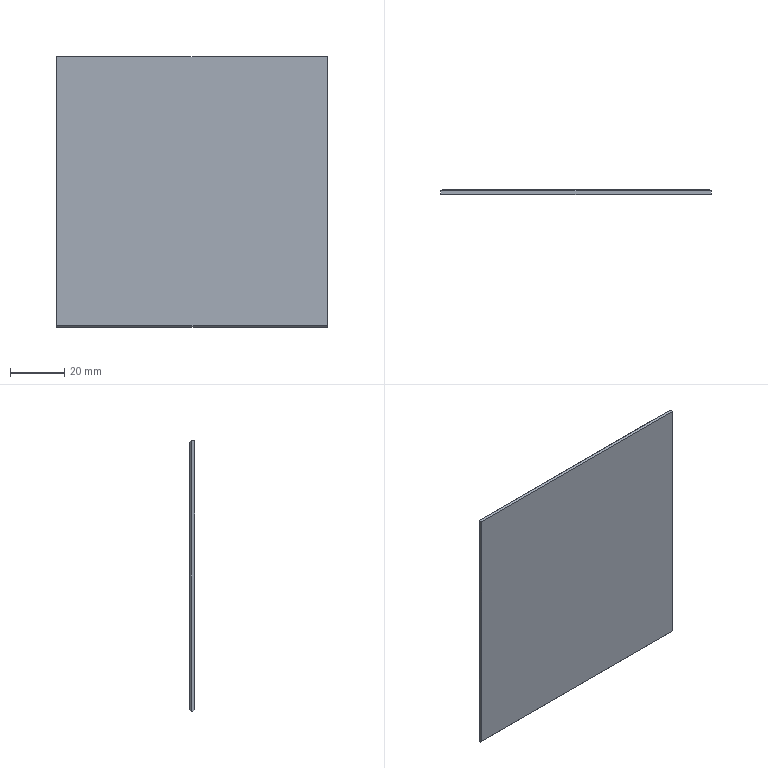Component | SolidWorks | PC-CAJ-P08-1_PM-CAJ-P60-1 | 1 solid | 11 faces | box 100 x 1.9 x 100 mm | volume 18910 mm3 | plane 11 | material Plain Carbon Steel
STEP:
#1=COLOUR_RGB('',0.7922,0.8196,0.9333);
#2=FILL_AREA_STYLE_COLOUR('',#1);
#3=FILL_AREA_STYLE('',(#2));
#4=SURFACE_STYLE_FILL_AREA(#3);
#5=SURFACE_SIDE_STYLE('',(#4));
#6=SURFACE_STYLE_USAGE(.BOTH.,#5);
#7=PRESENTATION_STYLE_ASSIGNMENT((#6));
#8=CARTESIAN_POINT('',(13.181,-26.622,8.976));
#9=VERTEX_POINT('',#8);
#10=CARTESIAN_POINT('',(13.181,-26.622,5.063));
#11=VERTEX_POINT('',#10);
#12=CARTESIAN_POINT('',(13.181,-26.622,7.008));
#13=DIRECTION('',(-0.,-0.,-1.));
#14=VECTOR('',#13,39.37);
#15=LINE('',#12,#14);
#16=EDGE_CURVE('',#9,#11,#15,.T.);
#17=ORIENTED_EDGE('',*,*,#16,.T.);
#18=CARTESIAN_POINT('',(13.181,-26.598,5.039));
#19=VERTEX_POINT('',#18);
#20=CARTESIAN_POINT('',(13.181,-28.579,7.02));
#21=DIRECTION('',(0.,0.7071,-0.7071));
#22=VECTOR('',#21,39.37);
#23=LINE('',#20,#22);
#24=EDGE_CURVE('',#11,#19,#23,.T.);
#25=ORIENTED_EDGE('',*,*,#24,.T.);
#26=CARTESIAN_POINT('',(13.181,-26.571,5.039));
#27=VERTEX_POINT('',#26);
#28=CARTESIAN_POINT('',(13.181,-26.585,5.039));
#29=DIRECTION('',(0.,1.,-0.));
#30=VECTOR('',#29,39.37);
#31=LINE('',#28,#30);
#32=EDGE_CURVE('',#19,#27,#31,.T.);
#33=ORIENTED_EDGE('',*,*,#32,.T.);
#34=CARTESIAN_POINT('',(13.181,-26.571,8.976));
#35=VERTEX_POINT('',#34);
#36=CARTESIAN_POINT('',(13.181,-26.571,8.976));
#37=DIRECTION('',(0.,0.,1.));
#38=VECTOR('',#37,39.37);
#39=LINE('',#36,#38);
#40=EDGE_CURVE('',#27,#35,#39,.T.);
#41=ORIENTED_EDGE('',*,*,#40,.T.);
#42=CARTESIAN_POINT('',(13.181,-26.585,8.976));
#43=DIRECTION('',(-0.,-1.,0.));
#44=VECTOR('',#43,39.37);
#45=LINE('',#42,#44);
#46=EDGE_CURVE('',#35,#9,#45,.T.);
#47=ORIENTED_EDGE('',*,*,#46,.T.);
#48=EDGE_LOOP('',(#17,#25,#33,#41,#47));
#49=FACE_OUTER_BOUND('',#48,.T.);
#50=CARTESIAN_POINT('',(13.181,-26.622,8.976));
#51=DIRECTION('',(1.,-0.,-0.));
#52=DIRECTION('',(-0.,-0.,-1.));
#53=AXIS2_PLACEMENT_3D('',#50,#51,#52);
#54=PLANE('',#53);
#55=ADVANCED_FACE('',(#49),#54,.T.);
#56=ORIENTED_EDGE('',*,*,#32,.F.);
#57=CARTESIAN_POINT('',(9.244,-26.598,5.039));
#58=VERTEX_POINT('',#57);
#59=CARTESIAN_POINT('',(13.181,-26.598,5.039));
#60=DIRECTION('',(-1.,0.,0.));
#61=VECTOR('',#60,39.37);
#62=LINE('',#59,#61);
#63=EDGE_CURVE('',#19,#58,#62,.T.);
#64=ORIENTED_EDGE('',*,*,#63,.T.);
#65=CARTESIAN_POINT('',(9.244,-26.571,5.039));
#66=VERTEX_POINT('',#65);
#67=CARTESIAN_POINT('',(9.244,-26.585,5.039));
#68=DIRECTION('',(0.,1.,-0.));
#69=VECTOR('',#68,39.37);
#70=LINE('',#67,#69);
#71=EDGE_CURVE('',#58,#66,#70,.T.);
#72=ORIENTED_EDGE('',*,*,#71,.T.);
#73=CARTESIAN_POINT('',(13.181,-26.571,5.039));
#74=DIRECTION('',(1.,-0.,-0.));
#75=VECTOR('',#74,39.37);
#76=LINE('',#73,#75);
#77=EDGE_CURVE('',#66,#27,#76,.T.);
#78=ORIENTED_EDGE('',*,*,#77,.T.);
#79=EDGE_LOOP('',(#56,#64,#72,#78));
#80=FACE_OUTER_BOUND('',#79,.T.);
#81=CARTESIAN_POINT('',(13.181,-26.622,5.039));
#82=DIRECTION('',(-0.,-0.,-1.));
#83=DIRECTION('',(-1.,0.,0.));
#84=AXIS2_PLACEMENT_3D('',#81,#82,#83);
#85=PLANE('',#84);
#86=ADVANCED_FACE('',(#80),#85,.T.);
#87=CARTESIAN_POINT('',(9.244,-26.622,8.976));
#88=VERTEX_POINT('',#87);
#89=CARTESIAN_POINT('',(9.244,-26.622,5.063));
#90=VERTEX_POINT('',#89);
#91=CARTESIAN_POINT('',(9.244,-26.622,7.008));
#92=DIRECTION('',(-0.,-0.,-1.));
#93=VECTOR('',#92,39.37);
#94=LINE('',#91,#93);
#95=EDGE_CURVE('',#88,#90,#94,.T.);
#96=ORIENTED_EDGE('',*,*,#95,.T.);
#97=CARTESIAN_POINT('',(13.181,-26.622,5.063));
#98=DIRECTION('',(1.,-0.,-0.));
#99=VECTOR('',#98,39.37);
#100=LINE('',#97,#99);
#101=EDGE_CURVE('',#90,#11,#100,.T.);
#102=ORIENTED_EDGE('',*,*,#101,.T.);
#103=ORIENTED_EDGE('',*,*,#16,.F.);
#104=CARTESIAN_POINT('',(11.213,-26.622,8.976));
#105=DIRECTION('',(-1.,0.,0.));
#106=VECTOR('',#105,39.37);
#107=LINE('',#104,#106);
#108=EDGE_CURVE('',#9,#88,#107,.T.);
#109=ORIENTED_EDGE('',*,*,#108,.T.);
#110=EDGE_LOOP('',(#96,#102,#103,#109));
#111=FACE_OUTER_BOUND('',#110,.T.);
#112=CARTESIAN_POINT('',(13.181,-26.622,8.976));
#113=DIRECTION('',(-0.,-1.,0.));
#114=DIRECTION('',(-1.,0.,0.));
#115=AXIS2_PLACEMENT_3D('',#112,#113,#114);
#116=PLANE('',#115);
#117=ADVANCED_FACE('',(#111),#116,.T.);
#118=ORIENTED_EDGE('',*,*,#46,.F.);
#119=CARTESIAN_POINT('',(9.244,-26.571,8.976));
#120=VERTEX_POINT('',#119);
#121=CARTESIAN_POINT('',(9.244,-26.571,8.976));
#122=DIRECTION('',(-1.,0.,0.));
#123=VECTOR('',#122,39.37);
#124=LINE('',#121,#123);
#125=EDGE_CURVE('',#35,#120,#124,.T.);
#126=ORIENTED_EDGE('',*,*,#125,.T.);
#127=CARTESIAN_POINT('',(9.244,-26.585,8.976));
#128=DIRECTION('',(-0.,-1.,0.));
#129=VECTOR('',#128,39.37);
#130=LINE('',#127,#129);
#131=EDGE_CURVE('',#120,#88,#130,.T.);
#132=ORIENTED_EDGE('',*,*,#131,.T.);
#133=ORIENTED_EDGE('',*,*,#108,.F.);
#134=EDGE_LOOP('',(#118,#126,#132,#133));
#135=FACE_OUTER_BOUND('',#134,.T.);
#136=CARTESIAN_POINT('',(9.244,-26.622,8.976));
#137=DIRECTION('',(0.,0.,1.));
#138=DIRECTION('',(1.,-0.,-0.));
#139=AXIS2_PLACEMENT_3D('',#136,#137,#138);
#140=PLANE('',#139);
#141=ADVANCED_FACE('',(#135),#140,.T.);
#142=CARTESIAN_POINT('',(13.157,-26.547,5.063));
#143=VERTEX_POINT('',#142);
#144=CARTESIAN_POINT('',(9.268,-26.547,5.063));
#145=VERTEX_POINT('',#144);
#146=CARTESIAN_POINT('',(9.244,-26.547,5.063));
#147=DIRECTION('',(-1.,0.,0.));
#148=VECTOR('',#147,39.37);
#149=LINE('',#146,#148);
#150=EDGE_CURVE('',#143,#145,#149,.T.);
#151=ORIENTED_EDGE('',*,*,#150,.T.);
#152=CARTESIAN_POINT('',(9.268,-26.547,8.953));
#153=VERTEX_POINT('',#152);
#154=CARTESIAN_POINT('',(9.268,-26.547,8.976));
#155=DIRECTION('',(0.,0.,1.));
#156=VECTOR('',#155,39.37);
#157=LINE('',#154,#156);
#158=EDGE_CURVE('',#145,#153,#157,.T.);
#159=ORIENTED_EDGE('',*,*,#158,.T.);
#160=CARTESIAN_POINT('',(13.157,-26.547,8.953));
#161=VERTEX_POINT('',#160);
#162=CARTESIAN_POINT('',(9.244,-26.547,8.953));
#163=DIRECTION('',(1.,-0.,-0.));
#164=VECTOR('',#163,39.37);
#165=LINE('',#162,#164);
#166=EDGE_CURVE('',#153,#161,#165,.T.);
#167=ORIENTED_EDGE('',*,*,#166,.T.);
#168=CARTESIAN_POINT('',(13.157,-26.547,8.976));
#169=DIRECTION('',(-0.,-0.,-1.));
#170=VECTOR('',#169,39.37);
#171=LINE('',#168,#170);
#172=EDGE_CURVE('',#161,#143,#171,.T.);
#173=ORIENTED_EDGE('',*,*,#172,.T.);
#174=EDGE_LOOP('',(#151,#159,#167,#173));
#175=FACE_OUTER_BOUND('',#174,.T.);
#176=CARTESIAN_POINT('',(9.244,-26.547,8.976));
#177=DIRECTION('',(0.,1.,-0.));
#178=DIRECTION('',(1.,-0.,-0.));
#179=AXIS2_PLACEMENT_3D('',#176,#177,#178);
#180=PLANE('',#179);
#181=ADVANCED_FACE('',(#175),#180,.T.);
#182=ORIENTED_EDGE('',*,*,#131,.F.);
#183=CARTESIAN_POINT('',(9.244,-26.571,5.039));
#184=DIRECTION('',(-0.,-0.,-1.));
#185=VECTOR('',#184,39.37);
#186=LINE('',#183,#185);
#187=EDGE_CURVE('',#120,#66,#186,.T.);
#188=ORIENTED_EDGE('',*,*,#187,.T.);
#189=ORIENTED_EDGE('',*,*,#71,.F.);
#190=CARTESIAN_POINT('',(9.244,-26.61,5.051));
#191=DIRECTION('',(-0.,-0.7071,0.7071));
#192=VECTOR('',#191,39.37);
#193=LINE('',#190,#192);
#194=EDGE_CURVE('',#58,#90,#193,.T.);
#195=ORIENTED_EDGE('',*,*,#194,.T.);
#196=ORIENTED_EDGE('',*,*,#95,.F.);
#197=EDGE_LOOP('',(#182,#188,#189,#195,#196));
#198=FACE_OUTER_BOUND('',#197,.T.);
#199=CARTESIAN_POINT('',(9.244,-26.622,5.039));
#200=DIRECTION('',(-1.,0.,0.));
#201=DIRECTION('',(0.,0.,1.));
#202=AXIS2_PLACEMENT_3D('',#199,#200,#201);
#203=PLANE('',#202);
#204=ADVANCED_FACE('',(#198),#203,.T.);
#205=ORIENTED_EDGE('',*,*,#24,.F.);
#206=ORIENTED_EDGE('',*,*,#101,.F.);
#207=ORIENTED_EDGE('',*,*,#194,.F.);
#208=ORIENTED_EDGE('',*,*,#63,.F.);
#209=EDGE_LOOP('',(#205,#206,#207,#208));
#210=FACE_OUTER_BOUND('',#209,.T.);
#211=CARTESIAN_POINT('',(13.181,-26.598,5.039));
#212=DIRECTION('',(0.,0.7071,0.7071));
#213=DIRECTION('',(-1.,0.,0.));
#214=AXIS2_PLACEMENT_3D('',#211,#212,#213);
#215=PLANE('',#214);
#216=ADVANCED_FACE('',(#210),#215,.F.);
#217=ORIENTED_EDGE('',*,*,#77,.F.);
#218=CARTESIAN_POINT('',(10.556,-25.259,6.352));
#219=DIRECTION('',(0.5774,0.5774,0.5774));
#220=VECTOR('',#219,39.37);
#221=LINE('',#218,#220);
#222=EDGE_CURVE('',#66,#145,#221,.T.);
#223=ORIENTED_EDGE('',*,*,#222,.T.);
#224=ORIENTED_EDGE('',*,*,#150,.F.);
#225=CARTESIAN_POINT('',(13.181,-26.571,5.039));
#226=DIRECTION('',(-0.5774,0.5774,0.5774));
#227=VECTOR('',#226,39.37);
#228=LINE('',#225,#227);
#229=EDGE_CURVE('',#27,#143,#228,.T.);
#230=ORIENTED_EDGE('',*,*,#229,.F.);
#231=EDGE_LOOP('',(#217,#223,#224,#230));
#232=FACE_OUTER_BOUND('',#231,.T.);
#233=CARTESIAN_POINT('',(13.181,-26.571,5.039));
#234=DIRECTION('',(-0.,-0.7071,0.7071));
#235=DIRECTION('',(1.,-0.,-0.));
#236=AXIS2_PLACEMENT_3D('',#233,#234,#235);
#237=PLANE('',#236);
#238=ADVANCED_FACE('',(#232),#237,.F.);
#239=ORIENTED_EDGE('',*,*,#229,.T.);
#240=ORIENTED_EDGE('',*,*,#172,.F.);
#241=CARTESIAN_POINT('',(13.181,-26.571,8.976));
#242=DIRECTION('',(-0.5774,0.5774,-0.5774));
#243=VECTOR('',#242,39.37);
#244=LINE('',#241,#243);
#245=EDGE_CURVE('',#35,#161,#244,.T.);
#246=ORIENTED_EDGE('',*,*,#245,.F.);
#247=ORIENTED_EDGE('',*,*,#40,.F.);
#248=EDGE_LOOP('',(#239,#240,#246,#247));
#249=FACE_OUTER_BOUND('',#248,.T.);
#250=CARTESIAN_POINT('',(13.181,-26.571,8.976));
#251=DIRECTION('',(-0.7071,-0.7071,0.));
#252=DIRECTION('',(0.,0.,1.));
#253=AXIS2_PLACEMENT_3D('',#250,#251,#252);
#254=PLANE('',#253);
#255=ADVANCED_FACE('',(#249),#254,.F.);
#256=ORIENTED_EDGE('',*,*,#166,.F.);
#257=CARTESIAN_POINT('',(9.244,-26.571,8.976));
#258=DIRECTION('',(-0.5774,-0.5774,0.5774));
#259=VECTOR('',#258,39.37);
#260=LINE('',#257,#259);
#261=EDGE_CURVE('',#153,#120,#260,.T.);
#262=ORIENTED_EDGE('',*,*,#261,.T.);
#263=ORIENTED_EDGE('',*,*,#125,.F.);
#264=ORIENTED_EDGE('',*,*,#245,.T.);
#265=EDGE_LOOP('',(#256,#262,#263,#264));
#266=FACE_OUTER_BOUND('',#265,.T.);
#267=CARTESIAN_POINT('',(9.244,-26.571,8.976));
#268=DIRECTION('',(-0.,-0.7071,-0.7071));
#269=DIRECTION('',(-1.,0.,0.));
#270=AXIS2_PLACEMENT_3D('',#267,#268,#269);
#271=PLANE('',#270);
#272=ADVANCED_FACE('',(#266),#271,.F.);
#273=ORIENTED_EDGE('',*,*,#222,.F.);
#274=ORIENTED_EDGE('',*,*,#187,.F.);
#275=ORIENTED_EDGE('',*,*,#261,.F.);
#276=ORIENTED_EDGE('',*,*,#158,.F.);
#277=EDGE_LOOP('',(#273,#274,#275,#276));
#278=FACE_OUTER_BOUND('',#277,.T.);
#279=CARTESIAN_POINT('',(9.268,-26.547,8.976));
#280=DIRECTION('',(0.7071,-0.7071,0.));
#281=DIRECTION('',(0.,0.,1.));
#282=AXIS2_PLACEMENT_3D('',#279,#280,#281);
#283=PLANE('',#282);
#284=ADVANCED_FACE('',(#278),#283,.F.);
#285=CLOSED_SHELL('',(#55,#86,#117,#141,#181,#204,#216,#238,#255,#272,#284));
#286=MANIFOLD_SOLID_BREP('',#285);
#287=STYLED_ITEM('',(#7),#286);
#288=(LENGTH_UNIT()NAMED_UNIT(*)SI_UNIT($,.METRE.));
#289=LENGTH_MEASURE_WITH_UNIT(LENGTH_MEASURE(0.0254),#288);
#290=DIMENSIONAL_EXPONENTS(1.,0.,0.,0.,0.,0.,0.);
#291=(CONVERSION_BASED_UNIT('',#289)LENGTH_UNIT()NAMED_UNIT(#290));
#292=UNCERTAINTY_MEASURE_WITH_UNIT(LENGTH_MEASURE(0.00001),#291,'','');
#293=(NAMED_UNIT(*)PLANE_ANGLE_UNIT()SI_UNIT($,.RADIAN.));
#294=(NAMED_UNIT(*)SI_UNIT($,.STERADIAN.)SOLID_ANGLE_UNIT());
#295=(GEOMETRIC_REPRESENTATION_CONTEXT(3)GLOBAL_UNCERTAINTY_ASSIGNED_CONTEXT((#292))GLOBAL_UNIT_ASSIGNED_CONTEXT((#291,#293,#294))REPRESENTATION_CONTEXT('',''));
#296=MECHANICAL_DESIGN_GEOMETRIC_PRESENTATION_REPRESENTATION('',(#287),#295);
#297=PRESENTATION_LAYER_ASSIGNMENT('','',(#287));
#298=CARTESIAN_POINT('',(0.,0.,0.));
#299=DIRECTION('',(0.,0.,1.));
#300=DIRECTION('',(1.,0.,0.));
#301=AXIS2_PLACEMENT_3D('',#298,#299,#300);
#302=(LENGTH_UNIT()NAMED_UNIT(*)SI_UNIT($,.METRE.));
#303=LENGTH_MEASURE_WITH_UNIT(LENGTH_MEASURE(0.0254),#302);
#304=DIMENSIONAL_EXPONENTS(1.,0.,0.,0.,0.,0.,0.);
#305=(CONVERSION_BASED_UNIT('',#303)LENGTH_UNIT()NAMED_UNIT(#304));
#306=UNCERTAINTY_MEASURE_WITH_UNIT(LENGTH_MEASURE(0.00001),#305,'','');
#307=(NAMED_UNIT(*)PLANE_ANGLE_UNIT()SI_UNIT($,.RADIAN.));
#308=(NAMED_UNIT(*)SI_UNIT($,.STERADIAN.)SOLID_ANGLE_UNIT());
#309=(GEOMETRIC_REPRESENTATION_CONTEXT(3)GLOBAL_UNCERTAINTY_ASSIGNED_CONTEXT((#306))GLOBAL_UNIT_ASSIGNED_CONTEXT((#305,#307,#308))REPRESENTATION_CONTEXT('',''));
#310=ADVANCED_BREP_SHAPE_REPRESENTATION('',(#286,#301),#309);